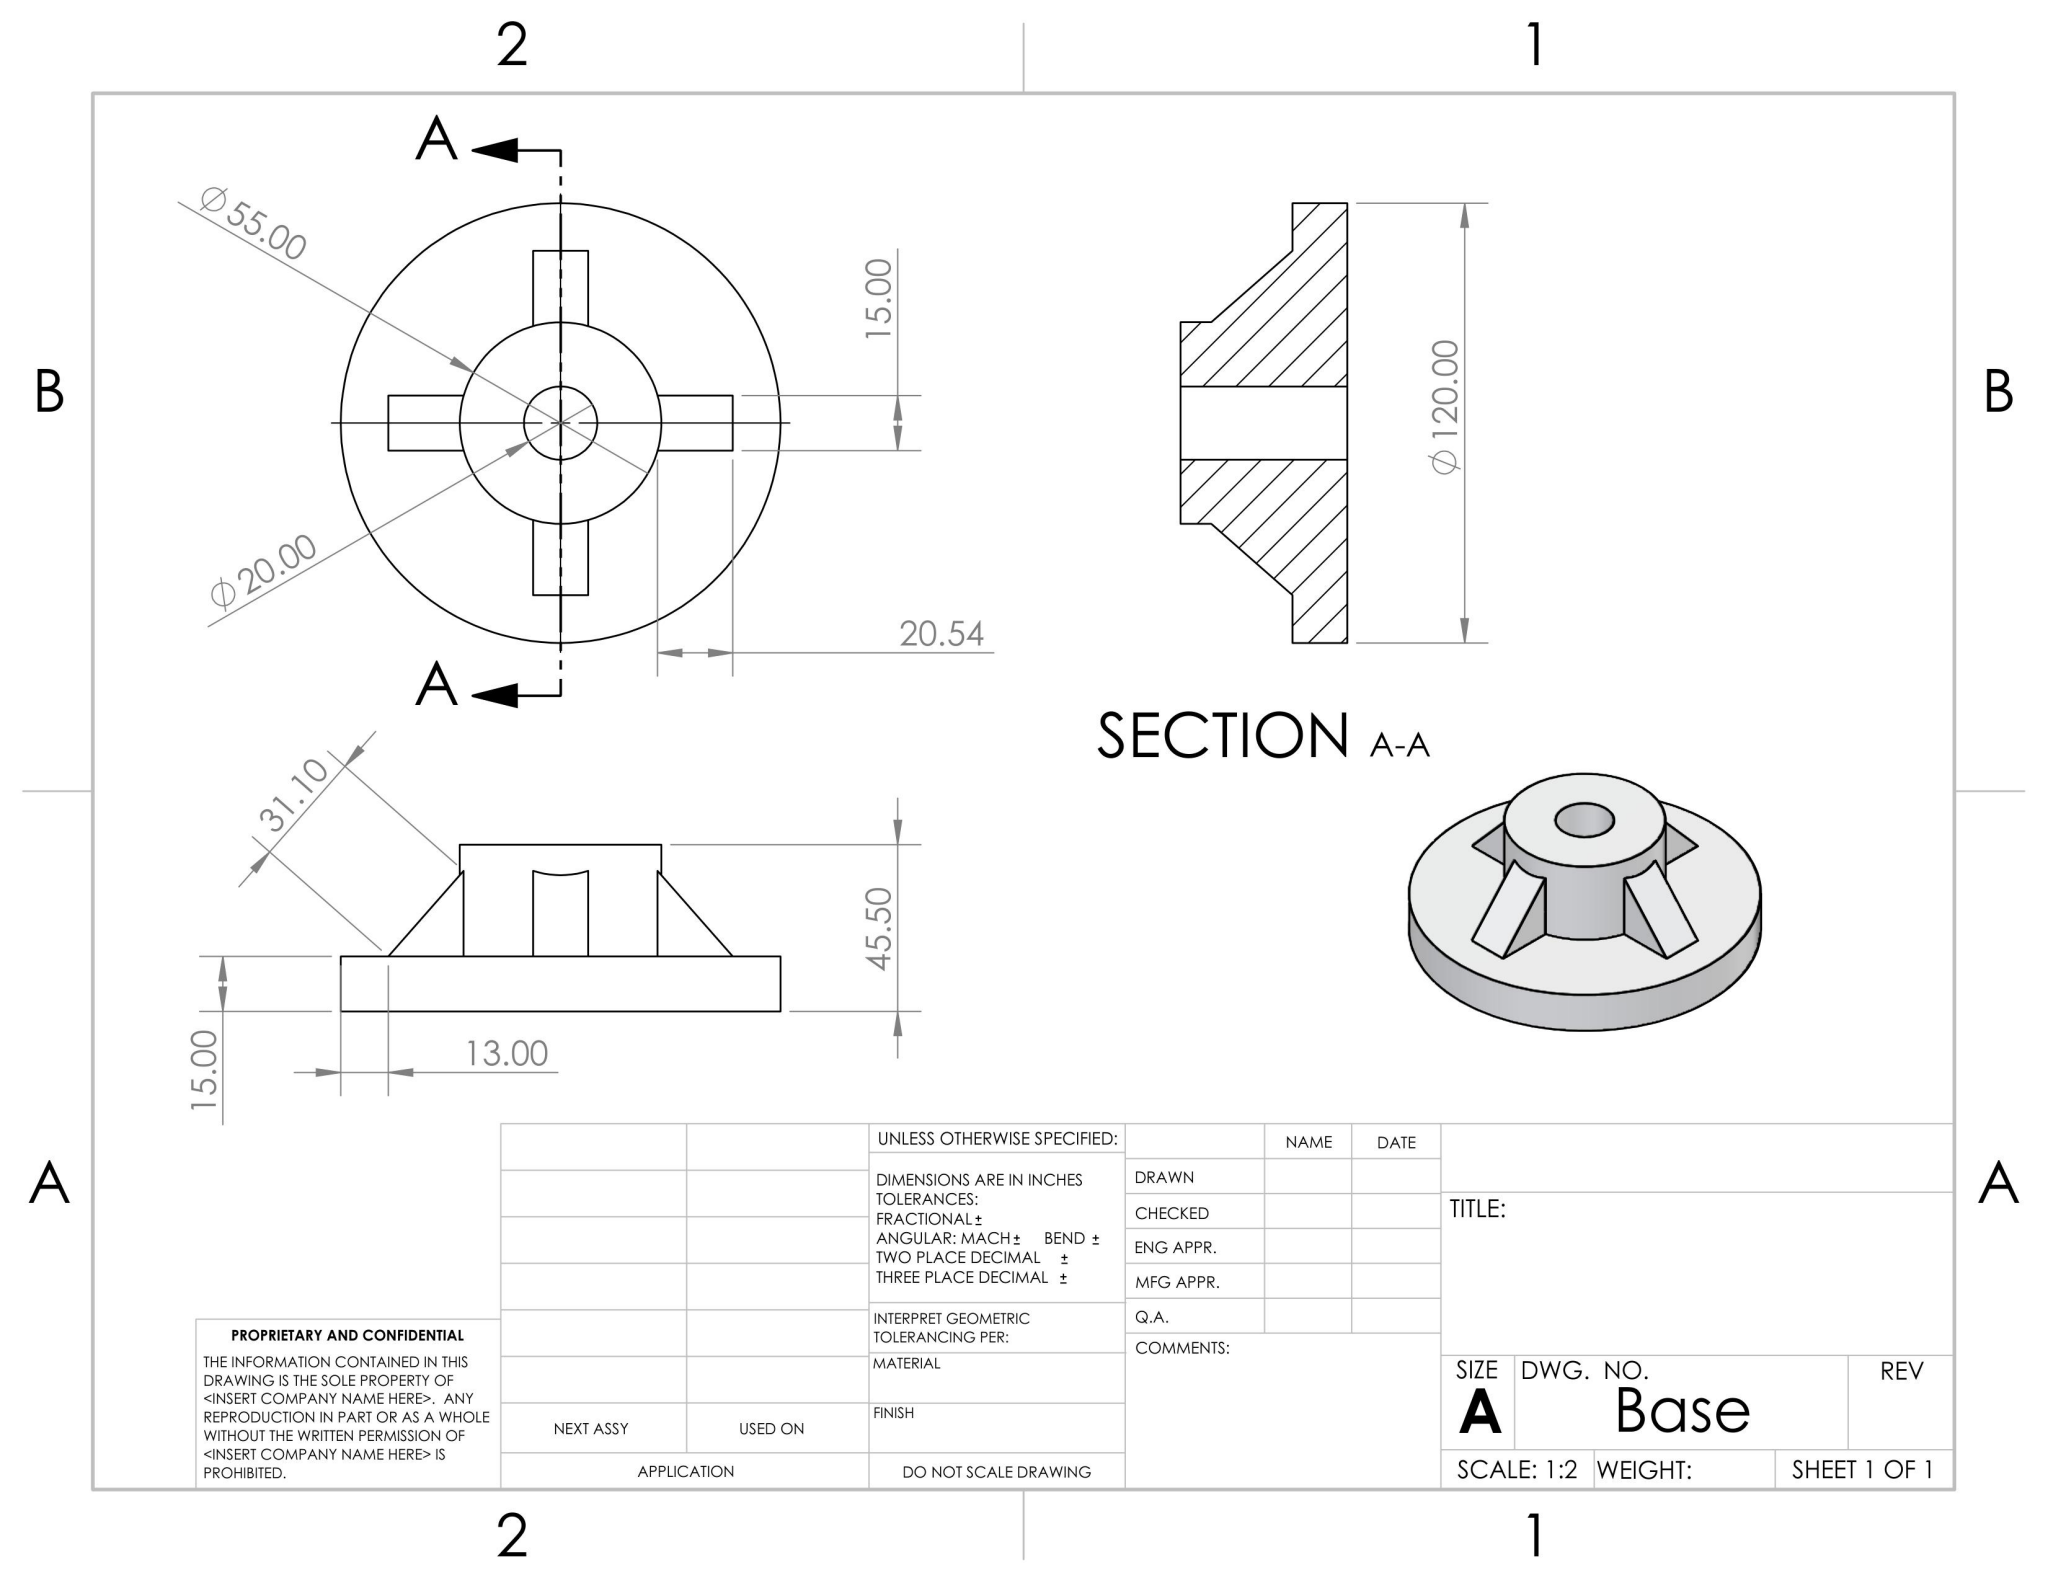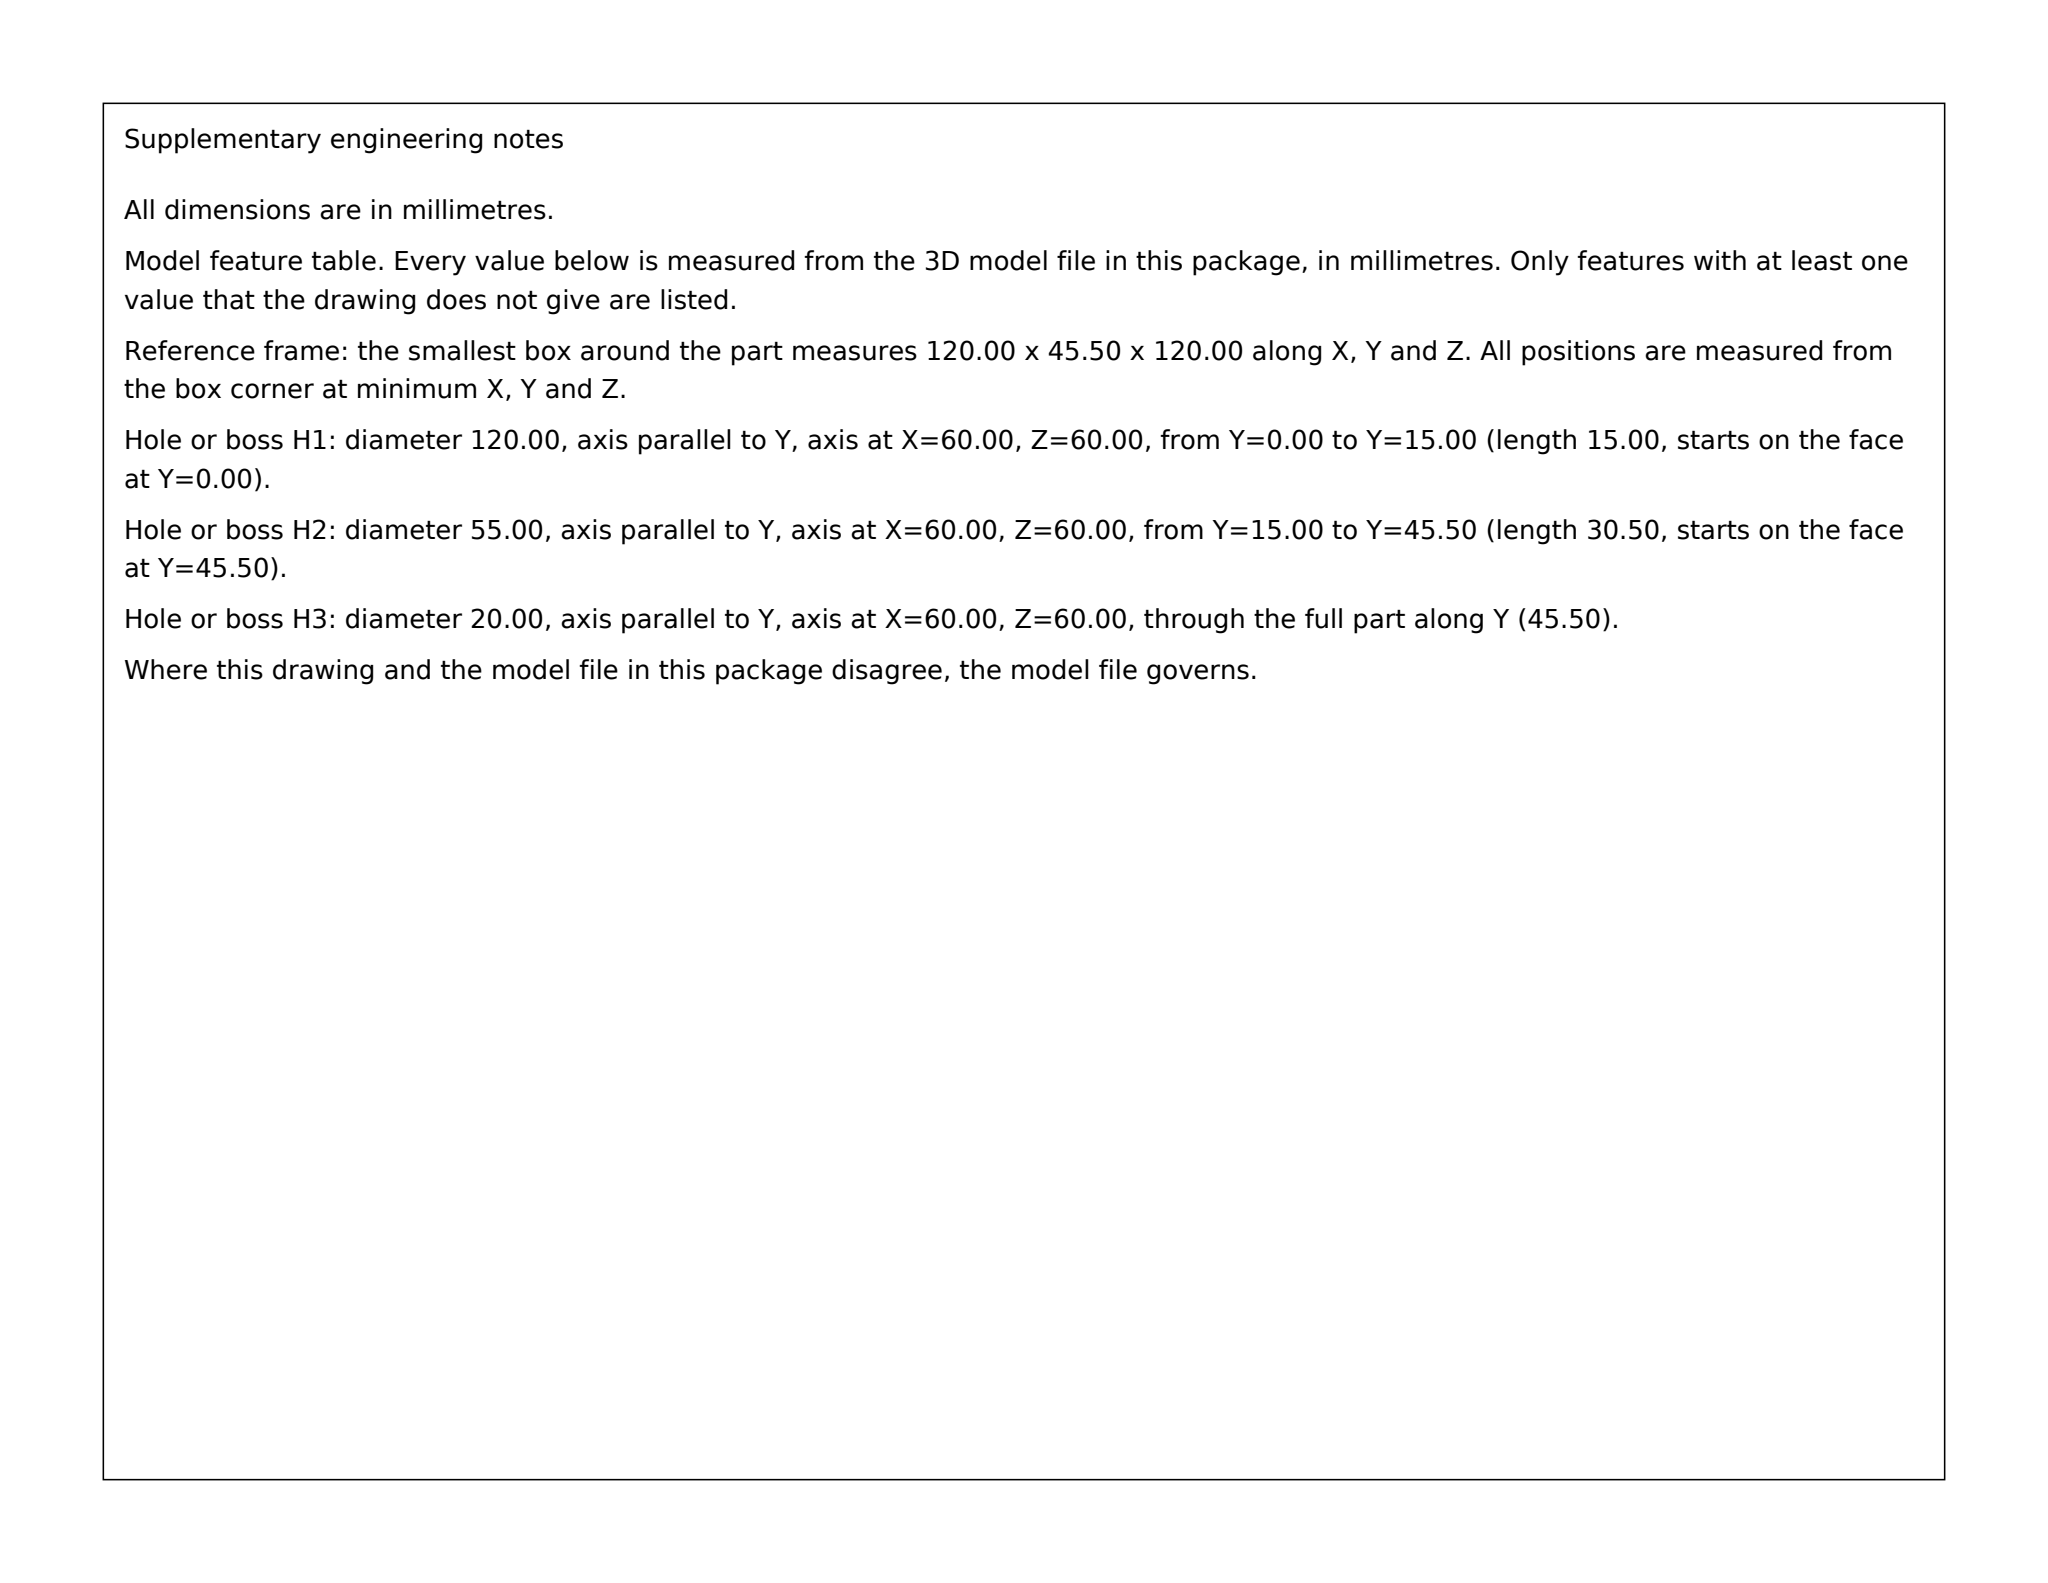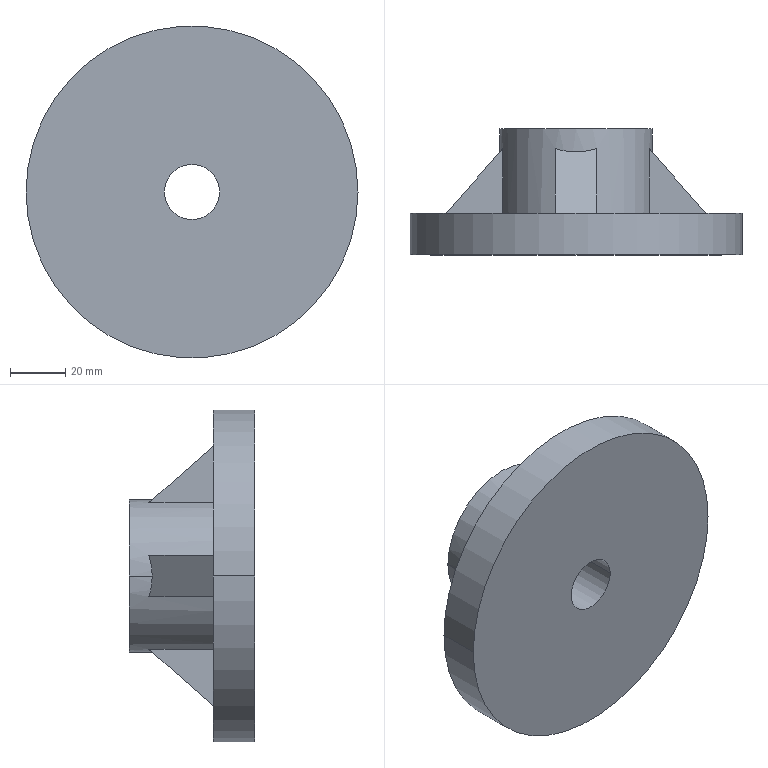Part | SolidWorks | mm | 1 solid | 21 faces | box 120 x 45.5 x 120 mm | volume 241243 mm3 | plane 15 | cylinder 6 | commonest cylinder face diameters 55 x2 120 x2 20 x2
build123d program:
from build123d import *

# Parameters (mm, degrees)
BOSS_EXTRUDE1_DEPTH             = 7.5
CIRPATTERN1_COUNT               = 4
SKETCH4_R                       = 27.5
SKETCH4_R_2                     = 10
BOSS_EXTRUDE2_DEPTH             = 0.5
BOSS_EXTRUDE2_DIRECTION_2_REACH = 98.047


with BuildPart() as part:
    # Sketch2 → Revolve1 (revolve)
    with BuildSketch(Plane.XY):
        Polygon((10, 22.5), (10, -22.5), (60, -22.5), (60, -7.5), (25, -7.5), (25, 22.5), align=None)
    revolve(axis=Axis((0, -22.5, 0), (0, 1, 0)))

    # Sketch3 → Boss-Extrude1 (add, symmetric)
    with BuildSketch(Plane.XY):
        Polygon((-47, -7.5), (-25, 17.5), (-17, 17.5), (-17, -10.5), (-47, -10.5), align=None)
    boss_extrude1 = extrude(amount=BOSS_EXTRUDE1_DEPTH, both=True)

    # CirPattern1: Boss-Extrude1 ×4 about axis
    cirpattern1_axis = Axis((0, 0, 0), (0, 1, 0))
    for i in range(1, CIRPATTERN1_COUNT):
        add(boss_extrude1.rotate(cirpattern1_axis, i * 360 / CIRPATTERN1_COUNT))

    # Sketch4 → Boss-Extrude2 (add)
    with BuildSketch(Plane(origin=(0, 22.5, 0), x_dir=(1, 0, 0), z_dir=(0, 1, 0))):
        with Locations(Location((0, 0, 0), (0, 0, 180))):
            Circle(SKETCH4_R)
        Circle(SKETCH4_R_2, mode=Mode.SUBTRACT)
    extrude(amount=BOSS_EXTRUDE2_DEPTH)

    # Boss-Extrude2 direction 2: up to this face of the body (flat: up to its plane)
    boss_extrude2_direction_2_end = Plane(part.part.faces().sort_by_distance((-58.303, -7.5, 0))[0])
    # Sketch4 → Boss-Extrude2 direction 2 (add, up to the picked face)
    with BuildSketch(Plane(origin=(0, 22.5, 0), x_dir=(1, 0, 0), z_dir=(0, 1, 0)), mode=Mode.PRIVATE) as boss_extrude2_direction_2_sk1:
        with Locations(Location((0, 0, 0), (0, 0, 180))):
            Circle(SKETCH4_R)
        Circle(SKETCH4_R_2, mode=Mode.SUBTRACT)
    boss_extrude2_direction_2_tool1 = split(extrude(boss_extrude2_direction_2_sk1.sketch, amount=-BOSS_EXTRUDE2_DIRECTION_2_REACH, mode=Mode.PRIVATE), bisect_by=boss_extrude2_direction_2_end, keep=Keep.BOTH, mode=Mode.PRIVATE)
    add(boss_extrude2_direction_2_tool1.solids().sort_by(Axis((26.722, 22.5, 0), (0, -1, 0)))[0])


solid = part.part
STEP:
#1=CARTESIAN_POINT('',(27.5,14.659,0.));
#2=VERTEX_POINT('',#1);
#3=CARTESIAN_POINT('',(26.458,15.844,7.5));
#4=VERTEX_POINT('',#3);
#5=CARTESIAN_POINT('',(27.5,14.659,0.));
#6=CARTESIAN_POINT('',(27.5,14.659,2.54));
#7=CARTESIAN_POINT('',(27.15,15.056,5.056));
#8=CARTESIAN_POINT('',(26.458,15.844,7.5));
#9=(BOUNDED_CURVE()B_SPLINE_CURVE(3,(#5,#6,#7,#8),.UNSPECIFIED.,.F.,.F.)B_SPLINE_CURVE_WITH_KNOTS((4,4),(3.142,3.418),.UNSPECIFIED.)CURVE()GEOMETRIC_REPRESENTATION_ITEM()RATIONAL_B_SPLINE_CURVE((1.,0.9937,0.9937,1.))REPRESENTATION_ITEM(''));
#10=EDGE_CURVE('',#2,#4,#9,.T.);
#11=ORIENTED_EDGE('',*,*,#10,.F.);
#12=CARTESIAN_POINT('',(27.5,23.,0.));
#13=VERTEX_POINT('',#12);
#14=CARTESIAN_POINT('',(27.5,-85.282,0.));
#15=DIRECTION('',(-0.,1.,0.));
#16=VECTOR('',#15,1000.);
#17=LINE('',#14,#16);
#18=EDGE_CURVE('',#2,#13,#17,.T.);
#19=ORIENTED_EDGE('',*,*,#18,.T.);
#20=CARTESIAN_POINT('',(-27.5,23.,0.));
#21=VERTEX_POINT('',#20);
#22=CARTESIAN_POINT('',(-0.,23.,0.));
#23=DIRECTION('',(-0.,1.,0.));
#24=DIRECTION('',(-1.,-0.,0.));
#25=AXIS2_PLACEMENT_3D('',#22,#23,#24);
#26=CIRCLE('',#25,27.5);
#27=EDGE_CURVE('',#21,#13,#26,.T.);
#28=ORIENTED_EDGE('',*,*,#27,.F.);
#29=CARTESIAN_POINT('',(-27.5,14.659,0.));
#30=VERTEX_POINT('',#29);
#31=CARTESIAN_POINT('',(-27.5,-85.282,0.));
#32=DIRECTION('',(-0.,1.,0.));
#33=VECTOR('',#32,1000.);
#34=LINE('',#31,#33);
#35=EDGE_CURVE('',#30,#21,#34,.T.);
#36=ORIENTED_EDGE('',*,*,#35,.F.);
#37=CARTESIAN_POINT('',(-26.458,15.844,7.5));
#38=VERTEX_POINT('',#37);
#39=CARTESIAN_POINT('',(-26.458,15.844,7.5));
#40=CARTESIAN_POINT('',(-27.15,15.056,5.056));
#41=CARTESIAN_POINT('',(-27.5,14.659,2.54));
#42=CARTESIAN_POINT('',(-27.5,14.659,0.));
#43=(BOUNDED_CURVE()B_SPLINE_CURVE(3,(#39,#40,#41,#42),.UNSPECIFIED.,.F.,.F.)B_SPLINE_CURVE_WITH_KNOTS((4,4),(2.865,3.142),.UNSPECIFIED.)CURVE()GEOMETRIC_REPRESENTATION_ITEM()RATIONAL_B_SPLINE_CURVE((1.,0.9937,0.9937,1.))REPRESENTATION_ITEM(''));
#44=EDGE_CURVE('',#38,#30,#43,.T.);
#45=ORIENTED_EDGE('',*,*,#44,.F.);
#46=CARTESIAN_POINT('',(-26.458,-7.5,7.5));
#47=VERTEX_POINT('',#46);
#48=CARTESIAN_POINT('',(-26.458,-85.282,7.5));
#49=DIRECTION('',(-0.,1.,0.));
#50=VECTOR('',#49,1000.);
#51=LINE('',#48,#50);
#52=EDGE_CURVE('',#47,#38,#51,.T.);
#53=ORIENTED_EDGE('',*,*,#52,.F.);
#54=CARTESIAN_POINT('',(-7.5,-7.5,26.458));
#55=VERTEX_POINT('',#54);
#56=CARTESIAN_POINT('',(0.,-7.5,0.));
#57=DIRECTION('',(0.,-1.,0.));
#58=DIRECTION('',(-1.,-0.,0.));
#59=AXIS2_PLACEMENT_3D('',#56,#57,#58);
#60=CIRCLE('',#59,27.5);
#61=EDGE_CURVE('',#55,#47,#60,.T.);
#62=ORIENTED_EDGE('',*,*,#61,.F.);
#63=CARTESIAN_POINT('',(-7.5,15.844,26.458));
#64=VERTEX_POINT('',#63);
#65=CARTESIAN_POINT('',(-7.5,-85.282,26.458));
#66=DIRECTION('',(-0.,1.,0.));
#67=VECTOR('',#66,1000.);
#68=LINE('',#65,#67);
#69=EDGE_CURVE('',#55,#64,#68,.T.);
#70=ORIENTED_EDGE('',*,*,#69,.T.);
#71=CARTESIAN_POINT('',(7.5,15.844,26.458));
#72=VERTEX_POINT('',#71);
#73=CARTESIAN_POINT('',(7.5,15.844,26.458));
#74=CARTESIAN_POINT('',(2.565,14.254,27.857));
#75=CARTESIAN_POINT('',(-2.565,14.254,27.857));
#76=CARTESIAN_POINT('',(-7.5,15.844,26.458));
#77=(BOUNDED_CURVE()B_SPLINE_CURVE(3,(#73,#74,#75,#76),.UNSPECIFIED.,.F.,.F.)B_SPLINE_CURVE_WITH_KNOTS((4,4),(2.865,3.418),.UNSPECIFIED.)CURVE()GEOMETRIC_REPRESENTATION_ITEM()RATIONAL_B_SPLINE_CURVE((1.,0.9747,0.9747,1.))REPRESENTATION_ITEM(''));
#78=EDGE_CURVE('',#72,#64,#77,.T.);
#79=ORIENTED_EDGE('',*,*,#78,.F.);
#80=CARTESIAN_POINT('',(7.5,-7.5,26.458));
#81=VERTEX_POINT('',#80);
#82=CARTESIAN_POINT('',(7.5,-85.282,26.458));
#83=DIRECTION('',(-0.,1.,0.));
#84=VECTOR('',#83,1000.);
#85=LINE('',#82,#84);
#86=EDGE_CURVE('',#81,#72,#85,.T.);
#87=ORIENTED_EDGE('',*,*,#86,.F.);
#88=CARTESIAN_POINT('',(26.458,-7.5,7.5));
#89=VERTEX_POINT('',#88);
#90=CARTESIAN_POINT('',(0.,-7.5,0.));
#91=DIRECTION('',(0.,-1.,0.));
#92=DIRECTION('',(-1.,-0.,0.));
#93=AXIS2_PLACEMENT_3D('',#90,#91,#92);
#94=CIRCLE('',#93,27.5);
#95=EDGE_CURVE('',#89,#81,#94,.T.);
#96=ORIENTED_EDGE('',*,*,#95,.F.);
#97=CARTESIAN_POINT('',(26.458,-85.282,7.5));
#98=DIRECTION('',(-0.,1.,0.));
#99=VECTOR('',#98,1000.);
#100=LINE('',#97,#99);
#101=EDGE_CURVE('',#89,#4,#100,.T.);
#102=ORIENTED_EDGE('',*,*,#101,.T.);
#103=EDGE_LOOP('',(#11,#19,#28,#36,#45,#53,#62,#70,#79,#87,#96,#102));
#104=FACE_OUTER_BOUND('',#103,.T.);
#105=CARTESIAN_POINT('',(0.,-85.282,0.));
#106=DIRECTION('',(-0.,1.,0.));
#107=DIRECTION('',(-1.,0.,0.));
#108=AXIS2_PLACEMENT_3D('',#105,#106,#107);
#109=CYLINDRICAL_SURFACE('',#108,27.5);
#110=ADVANCED_FACE('',(#104),#109,.T.);
#111=CARTESIAN_POINT('',(60.,-7.5,0.));
#112=VERTEX_POINT('',#111);
#113=CARTESIAN_POINT('',(-60.,-7.5,0.));
#114=VERTEX_POINT('',#113);
#115=CARTESIAN_POINT('',(-0.,-7.5,0.));
#116=DIRECTION('',(0.,-1.,0.));
#117=DIRECTION('',(1.,0.,0.));
#118=AXIS2_PLACEMENT_3D('',#115,#116,#117);
#119=CIRCLE('',#118,60.);
#120=EDGE_CURVE('',#112,#114,#119,.T.);
#121=ORIENTED_EDGE('',*,*,#120,.T.);
#122=CARTESIAN_POINT('',(-60.,-22.5,0.));
#123=VERTEX_POINT('',#122);
#124=CARTESIAN_POINT('',(-60.,-22.5,0.));
#125=DIRECTION('',(0.,-1.,0.));
#126=VECTOR('',#125,1000.);
#127=LINE('',#124,#126);
#128=EDGE_CURVE('',#114,#123,#127,.T.);
#129=ORIENTED_EDGE('',*,*,#128,.T.);
#130=CARTESIAN_POINT('',(60.,-22.5,0.));
#131=VERTEX_POINT('',#130);
#132=CARTESIAN_POINT('',(0.,-22.5,0.));
#133=DIRECTION('',(0.,-1.,0.));
#134=DIRECTION('',(1.,0.,0.));
#135=AXIS2_PLACEMENT_3D('',#132,#133,#134);
#136=CIRCLE('',#135,60.);
#137=EDGE_CURVE('',#131,#123,#136,.T.);
#138=ORIENTED_EDGE('',*,*,#137,.F.);
#139=CARTESIAN_POINT('',(60.,-22.5,0.));
#140=DIRECTION('',(0.,-1.,0.));
#141=VECTOR('',#140,1000.);
#142=LINE('',#139,#141);
#143=EDGE_CURVE('',#112,#131,#142,.T.);
#144=ORIENTED_EDGE('',*,*,#143,.F.);
#145=EDGE_LOOP('',(#121,#129,#138,#144));
#146=FACE_OUTER_BOUND('',#145,.T.);
#147=CARTESIAN_POINT('',(0.,-22.5,0.));
#148=DIRECTION('',(0.,-1.,0.));
#149=DIRECTION('',(1.,0.,0.));
#150=AXIS2_PLACEMENT_3D('',#147,#148,#149);
#151=CYLINDRICAL_SURFACE('',#150,60.);
#152=ADVANCED_FACE('',(#146),#151,.T.);
#153=CARTESIAN_POINT('',(10.,23.,0.));
#154=VERTEX_POINT('',#153);
#155=CARTESIAN_POINT('',(-10.,23.,0.));
#156=VERTEX_POINT('',#155);
#157=CARTESIAN_POINT('',(-0.,23.,0.));
#158=DIRECTION('',(-0.,1.,0.));
#159=DIRECTION('',(-1.,-0.,0.));
#160=AXIS2_PLACEMENT_3D('',#157,#158,#159);
#161=CIRCLE('',#160,10.);
#162=EDGE_CURVE('',#154,#156,#161,.T.);
#163=ORIENTED_EDGE('',*,*,#162,.T.);
#164=CARTESIAN_POINT('',(-10.,-22.5,0.));
#165=VERTEX_POINT('',#164);
#166=CARTESIAN_POINT('',(-10.,-22.5,0.));
#167=DIRECTION('',(0.,-1.,0.));
#168=VECTOR('',#167,1000.);
#169=LINE('',#166,#168);
#170=EDGE_CURVE('',#156,#165,#169,.T.);
#171=ORIENTED_EDGE('',*,*,#170,.T.);
#172=CARTESIAN_POINT('',(10.,-22.5,0.));
#173=VERTEX_POINT('',#172);
#174=CARTESIAN_POINT('',(-0.,-22.5,0.));
#175=DIRECTION('',(0.,-1.,0.));
#176=DIRECTION('',(1.,0.,0.));
#177=AXIS2_PLACEMENT_3D('',#174,#175,#176);
#178=CIRCLE('',#177,10.);
#179=EDGE_CURVE('',#165,#173,#178,.T.);
#180=ORIENTED_EDGE('',*,*,#179,.T.);
#181=CARTESIAN_POINT('',(10.,-22.5,0.));
#182=DIRECTION('',(0.,-1.,0.));
#183=VECTOR('',#182,1000.);
#184=LINE('',#181,#183);
#185=EDGE_CURVE('',#154,#173,#184,.T.);
#186=ORIENTED_EDGE('',*,*,#185,.F.);
#187=EDGE_LOOP('',(#163,#171,#180,#186));
#188=FACE_OUTER_BOUND('',#187,.T.);
#189=CARTESIAN_POINT('',(0.,-22.5,0.));
#190=DIRECTION('',(0.,-1.,0.));
#191=DIRECTION('',(1.,0.,0.));
#192=AXIS2_PLACEMENT_3D('',#189,#190,#191);
#193=CYLINDRICAL_SURFACE('',#192,10.);
#194=ADVANCED_FACE('',(#188),#193,.F.);
#195=ORIENTED_EDGE('',*,*,#120,.F.);
#196=CARTESIAN_POINT('',(-0.,-7.5,0.));
#197=DIRECTION('',(0.,-1.,0.));
#198=DIRECTION('',(1.,0.,0.));
#199=AXIS2_PLACEMENT_3D('',#196,#197,#198);
#200=CIRCLE('',#199,60.);
#201=EDGE_CURVE('',#114,#112,#200,.T.);
#202=ORIENTED_EDGE('',*,*,#201,.F.);
#203=EDGE_LOOP('',(#195,#202));
#204=FACE_OUTER_BOUND('',#203,.T.);
#205=CARTESIAN_POINT('',(-26.458,-7.5,-7.5));
#206=VERTEX_POINT('',#205);
#207=CARTESIAN_POINT('',(-47.,-7.5,-7.5));
#208=VERTEX_POINT('',#207);
#209=CARTESIAN_POINT('',(60.,-7.5,-7.5));
#210=DIRECTION('',(-1.,-0.,0.));
#211=VECTOR('',#210,1000.);
#212=LINE('',#209,#211);
#213=EDGE_CURVE('',#206,#208,#212,.T.);
#214=ORIENTED_EDGE('',*,*,#213,.F.);
#215=CARTESIAN_POINT('',(-7.5,-7.5,-26.458));
#216=VERTEX_POINT('',#215);
#217=CARTESIAN_POINT('',(0.,-7.5,0.));
#218=DIRECTION('',(0.,-1.,0.));
#219=DIRECTION('',(-1.,-0.,0.));
#220=AXIS2_PLACEMENT_3D('',#217,#218,#219);
#221=CIRCLE('',#220,27.5);
#222=EDGE_CURVE('',#206,#216,#221,.T.);
#223=ORIENTED_EDGE('',*,*,#222,.T.);
#224=CARTESIAN_POINT('',(-7.5,-7.5,-47.));
#225=VERTEX_POINT('',#224);
#226=CARTESIAN_POINT('',(-7.5,-7.5,-0.));
#227=DIRECTION('',(0.,0.,-1.));
#228=VECTOR('',#227,1000.);
#229=LINE('',#226,#228);
#230=EDGE_CURVE('',#216,#225,#229,.T.);
#231=ORIENTED_EDGE('',*,*,#230,.T.);
#232=CARTESIAN_POINT('',(7.5,-7.5,-47.));
#233=VERTEX_POINT('',#232);
#234=CARTESIAN_POINT('',(-7.5,-7.5,-47.));
#235=DIRECTION('',(1.,0.,0.));
#236=VECTOR('',#235,1000.);
#237=LINE('',#234,#236);
#238=EDGE_CURVE('',#225,#233,#237,.T.);
#239=ORIENTED_EDGE('',*,*,#238,.T.);
#240=CARTESIAN_POINT('',(7.5,-7.5,-26.458));
#241=VERTEX_POINT('',#240);
#242=CARTESIAN_POINT('',(7.5,-7.5,-0.));
#243=DIRECTION('',(0.,0.,-1.));
#244=VECTOR('',#243,1000.);
#245=LINE('',#242,#244);
#246=EDGE_CURVE('',#241,#233,#245,.T.);
#247=ORIENTED_EDGE('',*,*,#246,.F.);
#248=CARTESIAN_POINT('',(26.458,-7.5,-7.5));
#249=VERTEX_POINT('',#248);
#250=CARTESIAN_POINT('',(0.,-7.5,0.));
#251=DIRECTION('',(0.,-1.,0.));
#252=DIRECTION('',(-1.,-0.,0.));
#253=AXIS2_PLACEMENT_3D('',#250,#251,#252);
#254=CIRCLE('',#253,27.5);
#255=EDGE_CURVE('',#241,#249,#254,.T.);
#256=ORIENTED_EDGE('',*,*,#255,.T.);
#257=CARTESIAN_POINT('',(47.,-7.5,-7.5));
#258=VERTEX_POINT('',#257);
#259=CARTESIAN_POINT('',(60.,-7.5,-7.5));
#260=DIRECTION('',(1.,0.,0.));
#261=VECTOR('',#260,1000.);
#262=LINE('',#259,#261);
#263=EDGE_CURVE('',#249,#258,#262,.T.);
#264=ORIENTED_EDGE('',*,*,#263,.T.);
#265=CARTESIAN_POINT('',(47.,-7.5,7.5));
#266=VERTEX_POINT('',#265);
#267=CARTESIAN_POINT('',(47.,-7.5,-7.5));
#268=DIRECTION('',(0.,0.,1.));
#269=VECTOR('',#268,1000.);
#270=LINE('',#267,#269);
#271=EDGE_CURVE('',#258,#266,#270,.T.);
#272=ORIENTED_EDGE('',*,*,#271,.T.);
#273=CARTESIAN_POINT('',(60.,-7.5,7.5));
#274=DIRECTION('',(1.,0.,0.));
#275=VECTOR('',#274,1000.);
#276=LINE('',#273,#275);
#277=EDGE_CURVE('',#89,#266,#276,.T.);
#278=ORIENTED_EDGE('',*,*,#277,.F.);
#279=ORIENTED_EDGE('',*,*,#95,.T.);
#280=CARTESIAN_POINT('',(7.5,-7.5,47.));
#281=VERTEX_POINT('',#280);
#282=CARTESIAN_POINT('',(7.5,-7.5,-0.));
#283=DIRECTION('',(-0.,-0.,1.));
#284=VECTOR('',#283,1000.);
#285=LINE('',#282,#284);
#286=EDGE_CURVE('',#81,#281,#285,.T.);
#287=ORIENTED_EDGE('',*,*,#286,.T.);
#288=CARTESIAN_POINT('',(-7.5,-7.5,47.));
#289=VERTEX_POINT('',#288);
#290=CARTESIAN_POINT('',(7.5,-7.5,47.));
#291=DIRECTION('',(-1.,-0.,-0.));
#292=VECTOR('',#291,1000.);
#293=LINE('',#290,#292);
#294=EDGE_CURVE('',#281,#289,#293,.T.);
#295=ORIENTED_EDGE('',*,*,#294,.T.);
#296=CARTESIAN_POINT('',(-7.5,-7.5,-0.));
#297=DIRECTION('',(-0.,-0.,1.));
#298=VECTOR('',#297,1000.);
#299=LINE('',#296,#298);
#300=EDGE_CURVE('',#55,#289,#299,.T.);
#301=ORIENTED_EDGE('',*,*,#300,.F.);
#302=ORIENTED_EDGE('',*,*,#61,.T.);
#303=CARTESIAN_POINT('',(-47.,-7.5,7.5));
#304=VERTEX_POINT('',#303);
#305=CARTESIAN_POINT('',(60.,-7.5,7.5));
#306=DIRECTION('',(-1.,-0.,0.));
#307=VECTOR('',#306,1000.);
#308=LINE('',#305,#307);
#309=EDGE_CURVE('',#47,#304,#308,.T.);
#310=ORIENTED_EDGE('',*,*,#309,.T.);
#311=CARTESIAN_POINT('',(-47.,-7.5,7.5));
#312=DIRECTION('',(0.,0.,-1.));
#313=VECTOR('',#312,1000.);
#314=LINE('',#311,#313);
#315=EDGE_CURVE('',#304,#208,#314,.T.);
#316=ORIENTED_EDGE('',*,*,#315,.T.);
#317=EDGE_LOOP('',(#214,#223,#231,#239,#247,#256,#264,#272,#278,#279,#287,#295,#301,#302,#310,#316));
#318=FACE_BOUND('',#317,.T.);
#319=CARTESIAN_POINT('',(60.,-7.5,0.));
#320=DIRECTION('',(-0.,1.,0.));
#321=DIRECTION('',(-1.,-0.,0.));
#322=AXIS2_PLACEMENT_3D('',#319,#320,#321);
#323=PLANE('',#322);
#324=ADVANCED_FACE('',(#204,#318),#323,.T.);
#325=ORIENTED_EDGE('',*,*,#170,.F.);
#326=CARTESIAN_POINT('',(-0.,23.,0.));
#327=DIRECTION('',(-0.,1.,0.));
#328=DIRECTION('',(-1.,-0.,0.));
#329=AXIS2_PLACEMENT_3D('',#326,#327,#328);
#330=CIRCLE('',#329,10.);
#331=EDGE_CURVE('',#156,#154,#330,.T.);
#332=ORIENTED_EDGE('',*,*,#331,.T.);
#333=ORIENTED_EDGE('',*,*,#185,.T.);
#334=CARTESIAN_POINT('',(-0.,-22.5,0.));
#335=DIRECTION('',(0.,-1.,0.));
#336=DIRECTION('',(1.,0.,0.));
#337=AXIS2_PLACEMENT_3D('',#334,#335,#336);
#338=CIRCLE('',#337,10.);
#339=EDGE_CURVE('',#173,#165,#338,.T.);
#340=ORIENTED_EDGE('',*,*,#339,.T.);
#341=EDGE_LOOP('',(#325,#332,#333,#340));
#342=FACE_OUTER_BOUND('',#341,.T.);
#343=CARTESIAN_POINT('',(0.,-22.5,0.));
#344=DIRECTION('',(0.,-1.,0.));
#345=DIRECTION('',(1.,0.,0.));
#346=AXIS2_PLACEMENT_3D('',#343,#344,#345);
#347=CYLINDRICAL_SURFACE('',#346,10.);
#348=ADVANCED_FACE('',(#342),#347,.F.);
#349=ORIENTED_EDGE('',*,*,#137,.T.);
#350=CARTESIAN_POINT('',(0.,-22.5,0.));
#351=DIRECTION('',(0.,-1.,0.));
#352=DIRECTION('',(1.,0.,0.));
#353=AXIS2_PLACEMENT_3D('',#350,#351,#352);
#354=CIRCLE('',#353,60.);
#355=EDGE_CURVE('',#123,#131,#354,.T.);
#356=ORIENTED_EDGE('',*,*,#355,.T.);
#357=EDGE_LOOP('',(#349,#356));
#358=FACE_OUTER_BOUND('',#357,.T.);
#359=ORIENTED_EDGE('',*,*,#339,.F.);
#360=ORIENTED_EDGE('',*,*,#179,.F.);
#361=EDGE_LOOP('',(#359,#360));
#362=FACE_BOUND('',#361,.T.);
#363=CARTESIAN_POINT('',(10.,-22.5,0.));
#364=DIRECTION('',(0.,-1.,0.));
#365=DIRECTION('',(1.,0.,0.));
#366=AXIS2_PLACEMENT_3D('',#363,#364,#365);
#367=PLANE('',#366);
#368=ADVANCED_FACE('',(#358,#362),#367,.T.);
#369=ORIENTED_EDGE('',*,*,#128,.F.);
#370=ORIENTED_EDGE('',*,*,#201,.T.);
#371=ORIENTED_EDGE('',*,*,#143,.T.);
#372=ORIENTED_EDGE('',*,*,#355,.F.);
#373=EDGE_LOOP('',(#369,#370,#371,#372));
#374=FACE_OUTER_BOUND('',#373,.T.);
#375=CARTESIAN_POINT('',(0.,-22.5,0.));
#376=DIRECTION('',(0.,-1.,0.));
#377=DIRECTION('',(1.,0.,0.));
#378=AXIS2_PLACEMENT_3D('',#375,#376,#377);
#379=CYLINDRICAL_SURFACE('',#378,60.);
#380=ADVANCED_FACE('',(#374),#379,.T.);
#381=CARTESIAN_POINT('',(-47.,-7.5,7.5));
#382=DIRECTION('',(-0.6606,-0.7507,0.));
#383=VECTOR('',#382,1000.);
#384=LINE('',#381,#383);
#385=EDGE_CURVE('',#38,#304,#384,.T.);
#386=ORIENTED_EDGE('',*,*,#385,.F.);
#387=ORIENTED_EDGE('',*,*,#44,.T.);
#388=CARTESIAN_POINT('',(-26.458,15.844,-7.5));
#389=VERTEX_POINT('',#388);
#390=CARTESIAN_POINT('',(-27.5,14.659,0.));
#391=CARTESIAN_POINT('',(-27.5,14.659,-2.54));
#392=CARTESIAN_POINT('',(-27.15,15.056,-5.056));
#393=CARTESIAN_POINT('',(-26.458,15.844,-7.5));
#394=(BOUNDED_CURVE()B_SPLINE_CURVE(3,(#390,#391,#392,#393),.UNSPECIFIED.,.F.,.F.)B_SPLINE_CURVE_WITH_KNOTS((4,4),(3.142,3.418),.UNSPECIFIED.)CURVE()GEOMETRIC_REPRESENTATION_ITEM()RATIONAL_B_SPLINE_CURVE((1.,0.9937,0.9937,1.))REPRESENTATION_ITEM(''));
#395=EDGE_CURVE('',#30,#389,#394,.T.);
#396=ORIENTED_EDGE('',*,*,#395,.T.);
#397=CARTESIAN_POINT('',(-47.,-7.5,-7.5));
#398=DIRECTION('',(-0.6606,-0.7507,0.));
#399=VECTOR('',#398,1000.);
#400=LINE('',#397,#399);
#401=EDGE_CURVE('',#389,#208,#400,.T.);
#402=ORIENTED_EDGE('',*,*,#401,.T.);
#403=ORIENTED_EDGE('',*,*,#315,.F.);
#404=EDGE_LOOP('',(#386,#387,#396,#402,#403));
#405=FACE_OUTER_BOUND('',#404,.T.);
#406=CARTESIAN_POINT('',(-47.,-7.5,7.5));
#407=DIRECTION('',(0.7507,-0.6606,0.));
#408=DIRECTION('',(0.6606,0.7507,0.));
#409=AXIS2_PLACEMENT_3D('',#406,#407,#408);
#410=PLANE('',#409);
#411=ADVANCED_FACE('',(#405),#410,.F.);
#412=ORIENTED_EDGE('',*,*,#309,.F.);
#413=ORIENTED_EDGE('',*,*,#52,.T.);
#414=ORIENTED_EDGE('',*,*,#385,.T.);
#415=EDGE_LOOP('',(#412,#413,#414));
#416=FACE_OUTER_BOUND('',#415,.T.);
#417=CARTESIAN_POINT('',(0.,0.,7.5));
#418=DIRECTION('',(0.,0.,-1.));
#419=DIRECTION('',(-1.,0.,0.));
#420=AXIS2_PLACEMENT_3D('',#417,#418,#419);
#421=PLANE('',#420);
#422=ADVANCED_FACE('',(#416),#421,.F.);
#423=CARTESIAN_POINT('',(-26.458,-85.282,-7.5));
#424=DIRECTION('',(-0.,1.,0.));
#425=VECTOR('',#424,1000.);
#426=LINE('',#423,#425);
#427=EDGE_CURVE('',#206,#389,#426,.T.);
#428=ORIENTED_EDGE('',*,*,#427,.F.);
#429=ORIENTED_EDGE('',*,*,#213,.T.);
#430=ORIENTED_EDGE('',*,*,#401,.F.);
#431=EDGE_LOOP('',(#428,#429,#430));
#432=FACE_OUTER_BOUND('',#431,.T.);
#433=CARTESIAN_POINT('',(0.,0.,-7.5));
#434=DIRECTION('',(0.,0.,-1.));
#435=DIRECTION('',(-1.,0.,0.));
#436=AXIS2_PLACEMENT_3D('',#433,#434,#435);
#437=PLANE('',#436);
#438=ADVANCED_FACE('',(#432),#437,.T.);
#439=CARTESIAN_POINT('',(7.5,-7.5,47.));
#440=DIRECTION('',(-0.,-0.7507,0.6606));
#441=VECTOR('',#440,1000.);
#442=LINE('',#439,#441);
#443=EDGE_CURVE('',#72,#281,#442,.T.);
#444=ORIENTED_EDGE('',*,*,#443,.F.);
#445=ORIENTED_EDGE('',*,*,#78,.T.);
#446=CARTESIAN_POINT('',(-7.5,-7.5,47.));
#447=DIRECTION('',(-0.,-0.7507,0.6606));
#448=VECTOR('',#447,1000.);
#449=LINE('',#446,#448);
#450=EDGE_CURVE('',#64,#289,#449,.T.);
#451=ORIENTED_EDGE('',*,*,#450,.T.);
#452=ORIENTED_EDGE('',*,*,#294,.F.);
#453=EDGE_LOOP('',(#444,#445,#451,#452));
#454=FACE_OUTER_BOUND('',#453,.T.);
#455=CARTESIAN_POINT('',(7.5,-7.5,47.));
#456=DIRECTION('',(0.,-0.6606,-0.7507));
#457=DIRECTION('',(0.,0.7507,-0.6606));
#458=AXIS2_PLACEMENT_3D('',#455,#456,#457);
#459=PLANE('',#458);
#460=ADVANCED_FACE('',(#454),#459,.F.);
#461=ORIENTED_EDGE('',*,*,#286,.F.);
#462=ORIENTED_EDGE('',*,*,#86,.T.);
#463=ORIENTED_EDGE('',*,*,#443,.T.);
#464=EDGE_LOOP('',(#461,#462,#463));
#465=FACE_OUTER_BOUND('',#464,.T.);
#466=CARTESIAN_POINT('',(7.5,0.,0.));
#467=DIRECTION('',(-1.,-0.,-0.));
#468=DIRECTION('',(-0.,0.,1.));
#469=AXIS2_PLACEMENT_3D('',#466,#467,#468);
#470=PLANE('',#469);
#471=ADVANCED_FACE('',(#465),#470,.F.);
#472=ORIENTED_EDGE('',*,*,#69,.F.);
#473=ORIENTED_EDGE('',*,*,#300,.T.);
#474=ORIENTED_EDGE('',*,*,#450,.F.);
#475=EDGE_LOOP('',(#472,#473,#474));
#476=FACE_OUTER_BOUND('',#475,.T.);
#477=CARTESIAN_POINT('',(-7.5,-0.,-0.));
#478=DIRECTION('',(-1.,-0.,-0.));
#479=DIRECTION('',(-0.,0.,1.));
#480=AXIS2_PLACEMENT_3D('',#477,#478,#479);
#481=PLANE('',#480);
#482=ADVANCED_FACE('',(#476),#481,.T.);
#483=CARTESIAN_POINT('',(26.458,15.844,-7.5));
#484=VERTEX_POINT('',#483);
#485=CARTESIAN_POINT('',(47.,-7.5,-7.5));
#486=DIRECTION('',(0.6606,-0.7507,0.));
#487=VECTOR('',#486,1000.);
#488=LINE('',#485,#487);
#489=EDGE_CURVE('',#484,#258,#488,.T.);
#490=ORIENTED_EDGE('',*,*,#489,.F.);
#491=CARTESIAN_POINT('',(26.458,15.844,-7.5));
#492=CARTESIAN_POINT('',(27.15,15.056,-5.056));
#493=CARTESIAN_POINT('',(27.5,14.659,-2.54));
#494=CARTESIAN_POINT('',(27.5,14.659,0.));
#495=(BOUNDED_CURVE()B_SPLINE_CURVE(3,(#491,#492,#493,#494),.UNSPECIFIED.,.F.,.F.)B_SPLINE_CURVE_WITH_KNOTS((4,4),(2.865,3.142),.UNSPECIFIED.)CURVE()GEOMETRIC_REPRESENTATION_ITEM()RATIONAL_B_SPLINE_CURVE((1.,0.9937,0.9937,1.))REPRESENTATION_ITEM(''));
#496=EDGE_CURVE('',#484,#2,#495,.T.);
#497=ORIENTED_EDGE('',*,*,#496,.T.);
#498=ORIENTED_EDGE('',*,*,#10,.T.);
#499=CARTESIAN_POINT('',(47.,-7.5,7.5));
#500=DIRECTION('',(0.6606,-0.7507,0.));
#501=VECTOR('',#500,1000.);
#502=LINE('',#499,#501);
#503=EDGE_CURVE('',#4,#266,#502,.T.);
#504=ORIENTED_EDGE('',*,*,#503,.T.);
#505=ORIENTED_EDGE('',*,*,#271,.F.);
#506=EDGE_LOOP('',(#490,#497,#498,#504,#505));
#507=FACE_OUTER_BOUND('',#506,.T.);
#508=CARTESIAN_POINT('',(47.,-7.5,-7.5));
#509=DIRECTION('',(-0.7507,-0.6606,0.));
#510=DIRECTION('',(0.6606,-0.7507,0.));
#511=AXIS2_PLACEMENT_3D('',#508,#509,#510);
#512=PLANE('',#511);
#513=ADVANCED_FACE('',(#507),#512,.F.);
#514=ORIENTED_EDGE('',*,*,#263,.F.);
#515=CARTESIAN_POINT('',(26.458,-85.282,-7.5));
#516=DIRECTION('',(-0.,1.,0.));
#517=VECTOR('',#516,1000.);
#518=LINE('',#515,#517);
#519=EDGE_CURVE('',#249,#484,#518,.T.);
#520=ORIENTED_EDGE('',*,*,#519,.T.);
#521=ORIENTED_EDGE('',*,*,#489,.T.);
#522=EDGE_LOOP('',(#514,#520,#521));
#523=FACE_OUTER_BOUND('',#522,.T.);
#524=CARTESIAN_POINT('',(0.,0.,-7.5));
#525=DIRECTION('',(0.,0.,1.));
#526=DIRECTION('',(1.,0.,0.));
#527=AXIS2_PLACEMENT_3D('',#524,#525,#526);
#528=PLANE('',#527);
#529=ADVANCED_FACE('',(#523),#528,.F.);
#530=ORIENTED_EDGE('',*,*,#101,.F.);
#531=ORIENTED_EDGE('',*,*,#277,.T.);
#532=ORIENTED_EDGE('',*,*,#503,.F.);
#533=EDGE_LOOP('',(#530,#531,#532));
#534=FACE_OUTER_BOUND('',#533,.T.);
#535=CARTESIAN_POINT('',(0.,0.,7.5));
#536=DIRECTION('',(0.,0.,1.));
#537=DIRECTION('',(1.,0.,0.));
#538=AXIS2_PLACEMENT_3D('',#535,#536,#537);
#539=PLANE('',#538);
#540=ADVANCED_FACE('',(#534),#539,.T.);
#541=CARTESIAN_POINT('',(-7.5,15.844,-26.458));
#542=VERTEX_POINT('',#541);
#543=CARTESIAN_POINT('',(-7.5,-7.5,-47.));
#544=DIRECTION('',(0.,-0.7507,-0.6606));
#545=VECTOR('',#544,1000.);
#546=LINE('',#543,#545);
#547=EDGE_CURVE('',#542,#225,#546,.T.);
#548=ORIENTED_EDGE('',*,*,#547,.F.);
#549=CARTESIAN_POINT('',(7.5,15.844,-26.458));
#550=VERTEX_POINT('',#549);
#551=CARTESIAN_POINT('',(-7.5,15.844,-26.458));
#552=CARTESIAN_POINT('',(-2.565,14.254,-27.857));
#553=CARTESIAN_POINT('',(2.565,14.254,-27.857));
#554=CARTESIAN_POINT('',(7.5,15.844,-26.458));
#555=(BOUNDED_CURVE()B_SPLINE_CURVE(3,(#551,#552,#553,#554),.UNSPECIFIED.,.F.,.F.)B_SPLINE_CURVE_WITH_KNOTS((4,4),(2.865,3.418),.UNSPECIFIED.)CURVE()GEOMETRIC_REPRESENTATION_ITEM()RATIONAL_B_SPLINE_CURVE((1.,0.9747,0.9747,1.))REPRESENTATION_ITEM(''));
#556=EDGE_CURVE('',#542,#550,#555,.T.);
#557=ORIENTED_EDGE('',*,*,#556,.T.);
#558=CARTESIAN_POINT('',(7.5,-7.5,-47.));
#559=DIRECTION('',(0.,-0.7507,-0.6606));
#560=VECTOR('',#559,1000.);
#561=LINE('',#558,#560);
#562=EDGE_CURVE('',#550,#233,#561,.T.);
#563=ORIENTED_EDGE('',*,*,#562,.T.);
#564=ORIENTED_EDGE('',*,*,#238,.F.);
#565=EDGE_LOOP('',(#548,#557,#563,#564));
#566=FACE_OUTER_BOUND('',#565,.T.);
#567=CARTESIAN_POINT('',(-7.5,-7.5,-47.));
#568=DIRECTION('',(-0.,-0.6606,0.7507));
#569=DIRECTION('',(0.,-0.7507,-0.6606));
#570=AXIS2_PLACEMENT_3D('',#567,#568,#569);
#571=PLANE('',#570);
#572=ADVANCED_FACE('',(#566),#571,.F.);
#573=ORIENTED_EDGE('',*,*,#230,.F.);
#574=CARTESIAN_POINT('',(-7.5,-85.282,-26.458));
#575=DIRECTION('',(-0.,1.,0.));
#576=VECTOR('',#575,1000.);
#577=LINE('',#574,#576);
#578=EDGE_CURVE('',#216,#542,#577,.T.);
#579=ORIENTED_EDGE('',*,*,#578,.T.);
#580=ORIENTED_EDGE('',*,*,#547,.T.);
#581=EDGE_LOOP('',(#573,#579,#580));
#582=FACE_OUTER_BOUND('',#581,.T.);
#583=CARTESIAN_POINT('',(-7.5,-0.,-0.));
#584=DIRECTION('',(1.,0.,0.));
#585=DIRECTION('',(0.,0.,-1.));
#586=AXIS2_PLACEMENT_3D('',#583,#584,#585);
#587=PLANE('',#586);
#588=ADVANCED_FACE('',(#582),#587,.F.);
#589=CARTESIAN_POINT('',(7.5,-85.282,-26.458));
#590=DIRECTION('',(-0.,1.,0.));
#591=VECTOR('',#590,1000.);
#592=LINE('',#589,#591);
#593=EDGE_CURVE('',#241,#550,#592,.T.);
#594=ORIENTED_EDGE('',*,*,#593,.F.);
#595=ORIENTED_EDGE('',*,*,#246,.T.);
#596=ORIENTED_EDGE('',*,*,#562,.F.);
#597=EDGE_LOOP('',(#594,#595,#596));
#598=FACE_OUTER_BOUND('',#597,.T.);
#599=CARTESIAN_POINT('',(7.5,0.,0.));
#600=DIRECTION('',(1.,0.,0.));
#601=DIRECTION('',(0.,0.,-1.));
#602=AXIS2_PLACEMENT_3D('',#599,#600,#601);
#603=PLANE('',#602);
#604=ADVANCED_FACE('',(#598),#603,.T.);
#605=ORIENTED_EDGE('',*,*,#18,.F.);
#606=ORIENTED_EDGE('',*,*,#496,.F.);
#607=ORIENTED_EDGE('',*,*,#519,.F.);
#608=ORIENTED_EDGE('',*,*,#255,.F.);
#609=ORIENTED_EDGE('',*,*,#593,.T.);
#610=ORIENTED_EDGE('',*,*,#556,.F.);
#611=ORIENTED_EDGE('',*,*,#578,.F.);
#612=ORIENTED_EDGE('',*,*,#222,.F.);
#613=ORIENTED_EDGE('',*,*,#427,.T.);
#614=ORIENTED_EDGE('',*,*,#395,.F.);
#615=ORIENTED_EDGE('',*,*,#35,.T.);
#616=CARTESIAN_POINT('',(-0.,23.,0.));
#617=DIRECTION('',(-0.,1.,0.));
#618=DIRECTION('',(-1.,-0.,0.));
#619=AXIS2_PLACEMENT_3D('',#616,#617,#618);
#620=CIRCLE('',#619,27.5);
#621=EDGE_CURVE('',#13,#21,#620,.T.);
#622=ORIENTED_EDGE('',*,*,#621,.F.);
#623=EDGE_LOOP('',(#605,#606,#607,#608,#609,#610,#611,#612,#613,#614,#615,#622));
#624=FACE_OUTER_BOUND('',#623,.T.);
#625=CARTESIAN_POINT('',(0.,-85.282,0.));
#626=DIRECTION('',(-0.,1.,0.));
#627=DIRECTION('',(-1.,0.,0.));
#628=AXIS2_PLACEMENT_3D('',#625,#626,#627);
#629=CYLINDRICAL_SURFACE('',#628,27.5);
#630=ADVANCED_FACE('',(#624),#629,.T.);
#631=ORIENTED_EDGE('',*,*,#27,.T.);
#632=ORIENTED_EDGE('',*,*,#621,.T.);
#633=EDGE_LOOP('',(#631,#632));
#634=FACE_OUTER_BOUND('',#633,.T.);
#635=ORIENTED_EDGE('',*,*,#162,.F.);
#636=ORIENTED_EDGE('',*,*,#331,.F.);
#637=EDGE_LOOP('',(#635,#636));
#638=FACE_BOUND('',#637,.T.);
#639=CARTESIAN_POINT('',(-0.,23.,0.));
#640=DIRECTION('',(-0.,1.,0.));
#641=DIRECTION('',(-1.,-0.,0.));
#642=AXIS2_PLACEMENT_3D('',#639,#640,#641);
#643=PLANE('',#642);
#644=ADVANCED_FACE('',(#634,#638),#643,.T.);
#645=CLOSED_SHELL('',(#110,#152,#194,#324,#348,#368,#380,#411,#422,#438,#460,#471,#482,#513,#529,#540,#572,#588,#604,#630,#644));
#646=MANIFOLD_SOLID_BREP('',#645);
#647=CARTESIAN_POINT('',(0.,0.,0.));
#648=DIRECTION('',(0.,0.,1.));
#649=DIRECTION('',(1.,0.,0.));
#650=AXIS2_PLACEMENT_3D('',#647,#648,#649);
#651=(LENGTH_UNIT()NAMED_UNIT(*)SI_UNIT(.MILLI.,.METRE.));
#652=UNCERTAINTY_MEASURE_WITH_UNIT(LENGTH_MEASURE(0.00001),#651,'','');
#653=(NAMED_UNIT(*)PLANE_ANGLE_UNIT()SI_UNIT($,.RADIAN.));
#654=(NAMED_UNIT(*)SI_UNIT($,.STERADIAN.)SOLID_ANGLE_UNIT());
#655=(GEOMETRIC_REPRESENTATION_CONTEXT(3)GLOBAL_UNCERTAINTY_ASSIGNED_CONTEXT((#652))GLOBAL_UNIT_ASSIGNED_CONTEXT((#651,#653,#654))REPRESENTATION_CONTEXT('',''));
#656=ADVANCED_BREP_SHAPE_REPRESENTATION('',(#646,#650),#655);